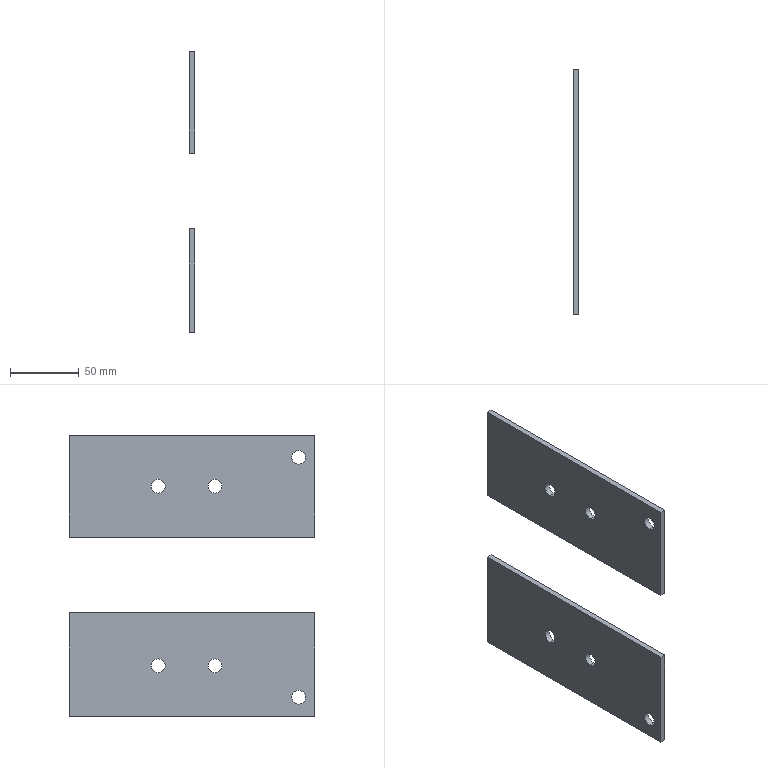Component | SolidWorks | Part2^Assembly2-1 | 2 solids | 24 faces | box 4 x 177.92 x 204 mm | volume 104314 mm3 | cylinder 12 | plane 12 | commonest cylinder face diameters 10 x12
STEP:
#1=COLOUR_RGB('',0.7922,0.8196,0.9333);
#2=FILL_AREA_STYLE_COLOUR('',#1);
#3=FILL_AREA_STYLE('',(#2));
#4=SURFACE_STYLE_FILL_AREA(#3);
#5=SURFACE_SIDE_STYLE('',(#4));
#6=SURFACE_STYLE_USAGE(.BOTH.,#5);
#7=PRESENTATION_STYLE_ASSIGNMENT((#6));
#8=CARTESIAN_POINT('',(6.188,14.393,-35.682));
#9=VERTEX_POINT('',#8);
#10=CARTESIAN_POINT('',(6.188,14.393,-36.076));
#11=VERTEX_POINT('',#10);
#12=CARTESIAN_POINT('',(6.188,14.393,-35.879));
#13=DIRECTION('',(1.,0.,0.));
#14=DIRECTION('',(0.,0.,-1.));
#15=AXIS2_PLACEMENT_3D('',#12,#13,#14);
#16=CIRCLE('',#15,0.1969);
#17=EDGE_CURVE('',#9,#11,#16,.T.);
#18=ORIENTED_EDGE('',*,*,#17,.F.);
#19=CARTESIAN_POINT('',(6.346,14.393,-35.682));
#20=VERTEX_POINT('',#19);
#21=CARTESIAN_POINT('',(2.133,14.393,-35.682));
#22=DIRECTION('',(1.,0.,0.));
#23=VECTOR('',#22,39.37);
#24=LINE('',#21,#23);
#25=EDGE_CURVE('',#9,#20,#24,.T.);
#26=ORIENTED_EDGE('',*,*,#25,.T.);
#27=CARTESIAN_POINT('',(6.346,14.393,-36.076));
#28=VERTEX_POINT('',#27);
#29=CARTESIAN_POINT('',(6.346,14.393,-35.879));
#30=DIRECTION('',(1.,0.,0.));
#31=DIRECTION('',(0.,0.,-1.));
#32=AXIS2_PLACEMENT_3D('',#29,#30,#31);
#33=CIRCLE('',#32,0.1969);
#34=EDGE_CURVE('',#20,#28,#33,.T.);
#35=ORIENTED_EDGE('',*,*,#34,.T.);
#36=CARTESIAN_POINT('',(2.133,14.393,-36.076));
#37=DIRECTION('',(1.,0.,0.));
#38=VECTOR('',#37,39.37);
#39=LINE('',#36,#38);
#40=EDGE_CURVE('',#11,#28,#39,.T.);
#41=ORIENTED_EDGE('',*,*,#40,.F.);
#42=EDGE_LOOP('',(#18,#26,#35,#41));
#43=FACE_OUTER_BOUND('',#42,.T.);
#44=CARTESIAN_POINT('',(2.133,14.393,-35.879));
#45=DIRECTION('',(1.,0.,0.));
#46=DIRECTION('',(0.,0.,-1.));
#47=AXIS2_PLACEMENT_3D('',#44,#45,#46);
#48=CYLINDRICAL_SURFACE('',#47,0.1969);
#49=ADVANCED_FACE('',(#43),#48,.F.);
#50=CARTESIAN_POINT('',(6.188,12.769,-35.682));
#51=VERTEX_POINT('',#50);
#52=CARTESIAN_POINT('',(6.188,12.769,-36.076));
#53=VERTEX_POINT('',#52);
#54=CARTESIAN_POINT('',(6.188,12.769,-35.879));
#55=DIRECTION('',(1.,0.,0.));
#56=DIRECTION('',(0.,0.,-1.));
#57=AXIS2_PLACEMENT_3D('',#54,#55,#56);
#58=CIRCLE('',#57,0.1969);
#59=EDGE_CURVE('',#51,#53,#58,.T.);
#60=ORIENTED_EDGE('',*,*,#59,.F.);
#61=CARTESIAN_POINT('',(6.346,12.769,-35.682));
#62=VERTEX_POINT('',#61);
#63=CARTESIAN_POINT('',(2.133,12.769,-35.682));
#64=DIRECTION('',(1.,0.,0.));
#65=VECTOR('',#64,39.37);
#66=LINE('',#63,#65);
#67=EDGE_CURVE('',#51,#62,#66,.T.);
#68=ORIENTED_EDGE('',*,*,#67,.T.);
#69=CARTESIAN_POINT('',(6.346,12.769,-36.076));
#70=VERTEX_POINT('',#69);
#71=CARTESIAN_POINT('',(6.346,12.769,-35.879));
#72=DIRECTION('',(1.,0.,0.));
#73=DIRECTION('',(0.,0.,-1.));
#74=AXIS2_PLACEMENT_3D('',#71,#72,#73);
#75=CIRCLE('',#74,0.1969);
#76=EDGE_CURVE('',#62,#70,#75,.T.);
#77=ORIENTED_EDGE('',*,*,#76,.T.);
#78=CARTESIAN_POINT('',(2.133,12.769,-36.076));
#79=DIRECTION('',(1.,0.,0.));
#80=VECTOR('',#79,39.37);
#81=LINE('',#78,#80);
#82=EDGE_CURVE('',#53,#70,#81,.T.);
#83=ORIENTED_EDGE('',*,*,#82,.F.);
#84=EDGE_LOOP('',(#60,#68,#77,#83));
#85=FACE_OUTER_BOUND('',#84,.T.);
#86=CARTESIAN_POINT('',(2.133,12.769,-35.879));
#87=DIRECTION('',(1.,0.,0.));
#88=DIRECTION('',(0.,0.,-1.));
#89=AXIS2_PLACEMENT_3D('',#86,#87,#88);
#90=CYLINDRICAL_SURFACE('',#89,0.1969);
#91=ADVANCED_FACE('',(#85),#90,.F.);
#92=CARTESIAN_POINT('',(6.188,10.383,-34.854));
#93=VERTEX_POINT('',#92);
#94=CARTESIAN_POINT('',(6.188,10.383,-35.248));
#95=VERTEX_POINT('',#94);
#96=CARTESIAN_POINT('',(6.188,10.383,-35.051));
#97=DIRECTION('',(1.,0.,0.));
#98=DIRECTION('',(0.,0.,-1.));
#99=AXIS2_PLACEMENT_3D('',#96,#97,#98);
#100=CIRCLE('',#99,0.1969);
#101=EDGE_CURVE('',#93,#95,#100,.T.);
#102=ORIENTED_EDGE('',*,*,#101,.F.);
#103=CARTESIAN_POINT('',(6.346,10.383,-34.854));
#104=VERTEX_POINT('',#103);
#105=CARTESIAN_POINT('',(6.188,10.383,-34.854));
#106=DIRECTION('',(1.,0.,0.));
#107=VECTOR('',#106,39.37);
#108=LINE('',#105,#107);
#109=EDGE_CURVE('',#93,#104,#108,.T.);
#110=ORIENTED_EDGE('',*,*,#109,.T.);
#111=CARTESIAN_POINT('',(6.346,10.383,-35.248));
#112=VERTEX_POINT('',#111);
#113=CARTESIAN_POINT('',(6.346,10.383,-35.051));
#114=DIRECTION('',(1.,0.,0.));
#115=DIRECTION('',(0.,0.,-1.));
#116=AXIS2_PLACEMENT_3D('',#113,#114,#115);
#117=CIRCLE('',#116,0.1969);
#118=EDGE_CURVE('',#104,#112,#117,.T.);
#119=ORIENTED_EDGE('',*,*,#118,.T.);
#120=CARTESIAN_POINT('',(6.188,10.383,-35.248));
#121=DIRECTION('',(1.,0.,0.));
#122=VECTOR('',#121,39.37);
#123=LINE('',#120,#122);
#124=EDGE_CURVE('',#95,#112,#123,.T.);
#125=ORIENTED_EDGE('',*,*,#124,.F.);
#126=EDGE_LOOP('',(#102,#110,#119,#125));
#127=FACE_OUTER_BOUND('',#126,.T.);
#128=CARTESIAN_POINT('',(6.188,10.383,-35.051));
#129=DIRECTION('',(1.,0.,0.));
#130=DIRECTION('',(0.,0.,-1.));
#131=AXIS2_PLACEMENT_3D('',#128,#129,#130);
#132=CYLINDRICAL_SURFACE('',#131,0.1969);
#133=ADVANCED_FACE('',(#127),#132,.F.);
#134=CARTESIAN_POINT('',(6.188,9.924,-34.426));
#135=VERTEX_POINT('',#134);
#136=CARTESIAN_POINT('',(6.188,9.924,-37.333));
#137=VERTEX_POINT('',#136);
#138=CARTESIAN_POINT('',(6.188,9.924,-34.426));
#139=DIRECTION('',(0.,0.,-1.));
#140=VECTOR('',#139,39.37);
#141=LINE('',#138,#140);
#142=EDGE_CURVE('',#135,#137,#141,.T.);
#143=ORIENTED_EDGE('',*,*,#142,.T.);
#144=CARTESIAN_POINT('',(6.346,9.924,-37.333));
#145=VERTEX_POINT('',#144);
#146=CARTESIAN_POINT('',(6.346,9.924,-37.333));
#147=DIRECTION('',(1.,0.,0.));
#148=VECTOR('',#147,39.37);
#149=LINE('',#146,#148);
#150=EDGE_CURVE('',#137,#145,#149,.T.);
#151=ORIENTED_EDGE('',*,*,#150,.T.);
#152=CARTESIAN_POINT('',(6.346,9.924,-34.426));
#153=VERTEX_POINT('',#152);
#154=CARTESIAN_POINT('',(6.346,9.924,-34.426));
#155=DIRECTION('',(0.,0.,-1.));
#156=VECTOR('',#155,39.37);
#157=LINE('',#154,#156);
#158=EDGE_CURVE('',#153,#145,#157,.T.);
#159=ORIENTED_EDGE('',*,*,#158,.F.);
#160=CARTESIAN_POINT('',(6.346,9.924,-34.426));
#161=DIRECTION('',(-1.,-0.,-0.));
#162=VECTOR('',#161,39.37);
#163=LINE('',#160,#162);
#164=EDGE_CURVE('',#153,#135,#163,.T.);
#165=ORIENTED_EDGE('',*,*,#164,.T.);
#166=EDGE_LOOP('',(#143,#151,#159,#165));
#167=FACE_OUTER_BOUND('',#166,.T.);
#168=CARTESIAN_POINT('',(6.346,9.924,-34.426));
#169=DIRECTION('',(-0.,1.,0.));
#170=DIRECTION('',(1.,0.,0.));
#171=AXIS2_PLACEMENT_3D('',#168,#169,#170);
#172=PLANE('',#171);
#173=ADVANCED_FACE('',(#167),#172,.F.);
#174=CARTESIAN_POINT('',(6.346,16.929,-37.333));
#175=VERTEX_POINT('',#174);
#176=CARTESIAN_POINT('',(6.346,16.929,-34.426));
#177=VERTEX_POINT('',#176);
#178=CARTESIAN_POINT('',(6.346,16.929,-34.426));
#179=DIRECTION('',(-0.,-0.,1.));
#180=VECTOR('',#179,39.37);
#181=LINE('',#178,#180);
#182=EDGE_CURVE('',#175,#177,#181,.T.);
#183=ORIENTED_EDGE('',*,*,#182,.F.);
#184=CARTESIAN_POINT('',(6.188,16.929,-37.333));
#185=VERTEX_POINT('',#184);
#186=CARTESIAN_POINT('',(6.346,16.929,-37.333));
#187=DIRECTION('',(-1.,-0.,-0.));
#188=VECTOR('',#187,39.37);
#189=LINE('',#186,#188);
#190=EDGE_CURVE('',#175,#185,#189,.T.);
#191=ORIENTED_EDGE('',*,*,#190,.T.);
#192=CARTESIAN_POINT('',(6.188,16.929,-34.426));
#193=VERTEX_POINT('',#192);
#194=CARTESIAN_POINT('',(6.188,16.929,-34.426));
#195=DIRECTION('',(-0.,-0.,1.));
#196=VECTOR('',#195,39.37);
#197=LINE('',#194,#196);
#198=EDGE_CURVE('',#185,#193,#197,.T.);
#199=ORIENTED_EDGE('',*,*,#198,.T.);
#200=CARTESIAN_POINT('',(6.346,16.929,-34.426));
#201=DIRECTION('',(-1.,-0.,-0.));
#202=VECTOR('',#201,39.37);
#203=LINE('',#200,#202);
#204=EDGE_CURVE('',#177,#193,#203,.T.);
#205=ORIENTED_EDGE('',*,*,#204,.F.);
#206=EDGE_LOOP('',(#183,#191,#199,#205));
#207=FACE_OUTER_BOUND('',#206,.T.);
#208=CARTESIAN_POINT('',(6.346,16.929,-34.426));
#209=DIRECTION('',(0.,-1.,0.));
#210=DIRECTION('',(-1.,-0.,-0.));
#211=AXIS2_PLACEMENT_3D('',#208,#209,#210);
#212=PLANE('',#211);
#213=ADVANCED_FACE('',(#207),#212,.F.);
#214=CARTESIAN_POINT('',(6.346,14.393,-35.879));
#215=DIRECTION('',(1.,0.,0.));
#216=DIRECTION('',(0.,0.,-1.));
#217=AXIS2_PLACEMENT_3D('',#214,#215,#216);
#218=CIRCLE('',#217,0.1969);
#219=EDGE_CURVE('',#28,#20,#218,.T.);
#220=ORIENTED_EDGE('',*,*,#219,.F.);
#221=ORIENTED_EDGE('',*,*,#34,.F.);
#222=EDGE_LOOP('',(#220,#221));
#223=FACE_BOUND('',#222,.T.);
#224=CARTESIAN_POINT('',(6.346,12.769,-35.879));
#225=DIRECTION('',(1.,0.,0.));
#226=DIRECTION('',(0.,0.,-1.));
#227=AXIS2_PLACEMENT_3D('',#224,#225,#226);
#228=CIRCLE('',#227,0.1969);
#229=EDGE_CURVE('',#70,#62,#228,.T.);
#230=ORIENTED_EDGE('',*,*,#229,.F.);
#231=ORIENTED_EDGE('',*,*,#76,.F.);
#232=EDGE_LOOP('',(#230,#231));
#233=FACE_BOUND('',#232,.T.);
#234=CARTESIAN_POINT('',(6.346,17.073,-37.333));
#235=DIRECTION('',(0.,-1.,0.));
#236=VECTOR('',#235,39.37);
#237=LINE('',#234,#236);
#238=EDGE_CURVE('',#175,#145,#237,.T.);
#239=ORIENTED_EDGE('',*,*,#238,.F.);
#240=ORIENTED_EDGE('',*,*,#182,.T.);
#241=CARTESIAN_POINT('',(6.346,16.929,-34.426));
#242=DIRECTION('',(0.,-1.,0.));
#243=VECTOR('',#242,39.37);
#244=LINE('',#241,#243);
#245=EDGE_CURVE('',#177,#153,#244,.T.);
#246=ORIENTED_EDGE('',*,*,#245,.T.);
#247=ORIENTED_EDGE('',*,*,#158,.T.);
#248=EDGE_LOOP('',(#239,#240,#246,#247));
#249=FACE_OUTER_BOUND('',#248,.T.);
#250=CARTESIAN_POINT('',(6.346,10.383,-35.051));
#251=DIRECTION('',(1.,0.,0.));
#252=DIRECTION('',(0.,0.,-1.));
#253=AXIS2_PLACEMENT_3D('',#250,#251,#252);
#254=CIRCLE('',#253,0.1969);
#255=EDGE_CURVE('',#112,#104,#254,.T.);
#256=ORIENTED_EDGE('',*,*,#255,.F.);
#257=ORIENTED_EDGE('',*,*,#118,.F.);
#258=EDGE_LOOP('',(#256,#257));
#259=FACE_BOUND('',#258,.T.);
#260=CARTESIAN_POINT('',(6.346,4.425,-14.841));
#261=DIRECTION('',(1.,0.,0.));
#262=DIRECTION('',(0.,0.,-1.));
#263=AXIS2_PLACEMENT_3D('',#260,#261,#262);
#264=PLANE('',#263);
#265=ADVANCED_FACE('',(#223,#233,#249,#259),#264,.T.);
#266=CARTESIAN_POINT('',(6.188,14.393,-35.879));
#267=DIRECTION('',(1.,0.,0.));
#268=DIRECTION('',(0.,0.,-1.));
#269=AXIS2_PLACEMENT_3D('',#266,#267,#268);
#270=CIRCLE('',#269,0.1969);
#271=EDGE_CURVE('',#11,#9,#270,.T.);
#272=ORIENTED_EDGE('',*,*,#271,.T.);
#273=ORIENTED_EDGE('',*,*,#17,.T.);
#274=EDGE_LOOP('',(#272,#273));
#275=FACE_BOUND('',#274,.T.);
#276=CARTESIAN_POINT('',(6.188,12.769,-35.879));
#277=DIRECTION('',(1.,0.,0.));
#278=DIRECTION('',(0.,0.,-1.));
#279=AXIS2_PLACEMENT_3D('',#276,#277,#278);
#280=CIRCLE('',#279,0.1969);
#281=EDGE_CURVE('',#53,#51,#280,.T.);
#282=ORIENTED_EDGE('',*,*,#281,.T.);
#283=ORIENTED_EDGE('',*,*,#59,.T.);
#284=EDGE_LOOP('',(#282,#283));
#285=FACE_BOUND('',#284,.T.);
#286=CARTESIAN_POINT('',(6.188,10.383,-35.051));
#287=DIRECTION('',(1.,0.,0.));
#288=DIRECTION('',(0.,0.,-1.));
#289=AXIS2_PLACEMENT_3D('',#286,#287,#288);
#290=CIRCLE('',#289,0.1969);
#291=EDGE_CURVE('',#95,#93,#290,.T.);
#292=ORIENTED_EDGE('',*,*,#291,.T.);
#293=ORIENTED_EDGE('',*,*,#101,.T.);
#294=EDGE_LOOP('',(#292,#293));
#295=FACE_BOUND('',#294,.T.);
#296=ORIENTED_EDGE('',*,*,#198,.F.);
#297=CARTESIAN_POINT('',(6.188,4.425,-37.333));
#298=DIRECTION('',(0.,-1.,0.));
#299=VECTOR('',#298,39.37);
#300=LINE('',#297,#299);
#301=EDGE_CURVE('',#185,#137,#300,.T.);
#302=ORIENTED_EDGE('',*,*,#301,.T.);
#303=ORIENTED_EDGE('',*,*,#142,.F.);
#304=CARTESIAN_POINT('',(6.188,16.929,-34.426));
#305=DIRECTION('',(0.,-1.,0.));
#306=VECTOR('',#305,39.37);
#307=LINE('',#304,#306);
#308=EDGE_CURVE('',#193,#135,#307,.T.);
#309=ORIENTED_EDGE('',*,*,#308,.F.);
#310=EDGE_LOOP('',(#296,#302,#303,#309));
#311=FACE_OUTER_BOUND('',#310,.T.);
#312=CARTESIAN_POINT('',(6.188,4.425,-14.841));
#313=DIRECTION('',(1.,0.,0.));
#314=DIRECTION('',(0.,0.,-1.));
#315=AXIS2_PLACEMENT_3D('',#312,#313,#314);
#316=PLANE('',#315);
#317=ADVANCED_FACE('',(#275,#285,#295,#311),#316,.F.);
#318=ORIENTED_EDGE('',*,*,#308,.T.);
#319=ORIENTED_EDGE('',*,*,#164,.F.);
#320=ORIENTED_EDGE('',*,*,#245,.F.);
#321=ORIENTED_EDGE('',*,*,#204,.T.);
#322=EDGE_LOOP('',(#318,#319,#320,#321));
#323=FACE_OUTER_BOUND('',#322,.T.);
#324=CARTESIAN_POINT('',(6.346,16.929,-34.426));
#325=DIRECTION('',(0.,0.,-1.));
#326=DIRECTION('',(-1.,-0.,-0.));
#327=AXIS2_PLACEMENT_3D('',#324,#325,#326);
#328=PLANE('',#327);
#329=ADVANCED_FACE('',(#323),#328,.F.);
#330=ORIENTED_EDGE('',*,*,#109,.F.);
#331=ORIENTED_EDGE('',*,*,#291,.F.);
#332=ORIENTED_EDGE('',*,*,#124,.T.);
#333=ORIENTED_EDGE('',*,*,#255,.T.);
#334=EDGE_LOOP('',(#330,#331,#332,#333));
#335=FACE_OUTER_BOUND('',#334,.T.);
#336=CARTESIAN_POINT('',(6.188,10.383,-35.051));
#337=DIRECTION('',(1.,0.,0.));
#338=DIRECTION('',(0.,0.,-1.));
#339=AXIS2_PLACEMENT_3D('',#336,#337,#338);
#340=CYLINDRICAL_SURFACE('',#339,0.1969);
#341=ADVANCED_FACE('',(#335),#340,.F.);
#342=ORIENTED_EDGE('',*,*,#301,.F.);
#343=ORIENTED_EDGE('',*,*,#190,.F.);
#344=ORIENTED_EDGE('',*,*,#238,.T.);
#345=ORIENTED_EDGE('',*,*,#150,.F.);
#346=EDGE_LOOP('',(#342,#343,#344,#345));
#347=FACE_OUTER_BOUND('',#346,.T.);
#348=CARTESIAN_POINT('',(2.133,17.073,-37.333));
#349=DIRECTION('',(-0.,-0.,1.));
#350=DIRECTION('',(1.,0.,0.));
#351=AXIS2_PLACEMENT_3D('',#348,#349,#350);
#352=PLANE('',#351);
#353=ADVANCED_FACE('',(#347),#352,.F.);
#354=ORIENTED_EDGE('',*,*,#67,.F.);
#355=ORIENTED_EDGE('',*,*,#281,.F.);
#356=ORIENTED_EDGE('',*,*,#82,.T.);
#357=ORIENTED_EDGE('',*,*,#229,.T.);
#358=EDGE_LOOP('',(#354,#355,#356,#357));
#359=FACE_OUTER_BOUND('',#358,.T.);
#360=CARTESIAN_POINT('',(2.133,12.769,-35.879));
#361=DIRECTION('',(1.,0.,0.));
#362=DIRECTION('',(0.,0.,-1.));
#363=AXIS2_PLACEMENT_3D('',#360,#361,#362);
#364=CYLINDRICAL_SURFACE('',#363,0.1969);
#365=ADVANCED_FACE('',(#359),#364,.F.);
#366=ORIENTED_EDGE('',*,*,#25,.F.);
#367=ORIENTED_EDGE('',*,*,#271,.F.);
#368=ORIENTED_EDGE('',*,*,#40,.T.);
#369=ORIENTED_EDGE('',*,*,#219,.T.);
#370=EDGE_LOOP('',(#366,#367,#368,#369));
#371=FACE_OUTER_BOUND('',#370,.T.);
#372=CARTESIAN_POINT('',(2.133,14.393,-35.879));
#373=DIRECTION('',(1.,0.,0.));
#374=DIRECTION('',(0.,0.,-1.));
#375=AXIS2_PLACEMENT_3D('',#372,#373,#374);
#376=CYLINDRICAL_SURFACE('',#375,0.1969);
#377=ADVANCED_FACE('',(#371),#376,.F.);
#378=CLOSED_SHELL('',(#49,#91,#133,#173,#213,#265,#317,#329,#341,#353,#365,#377));
#379=MANIFOLD_SOLID_BREP('',#378);
#380=STYLED_ITEM('',(#7),#379);
#381=(LENGTH_UNIT()NAMED_UNIT(*)SI_UNIT($,.METRE.));
#382=LENGTH_MEASURE_WITH_UNIT(LENGTH_MEASURE(0.0254),#381);
#383=DIMENSIONAL_EXPONENTS(1.,0.,0.,0.,0.,0.,0.);
#384=(CONVERSION_BASED_UNIT('',#382)LENGTH_UNIT()NAMED_UNIT(#383));
#385=UNCERTAINTY_MEASURE_WITH_UNIT(LENGTH_MEASURE(0.00001),#384,'','');
#386=(NAMED_UNIT(*)PLANE_ANGLE_UNIT()SI_UNIT($,.RADIAN.));
#387=(NAMED_UNIT(*)SI_UNIT($,.STERADIAN.)SOLID_ANGLE_UNIT());
#388=(GEOMETRIC_REPRESENTATION_CONTEXT(3)GLOBAL_UNCERTAINTY_ASSIGNED_CONTEXT((#385))GLOBAL_UNIT_ASSIGNED_CONTEXT((#384,#386,#387))REPRESENTATION_CONTEXT('',''));
#389=MECHANICAL_DESIGN_GEOMETRIC_PRESENTATION_REPRESENTATION('',(#380),#388);
#390=PRESENTATION_LAYER_ASSIGNMENT('','',(#380));
#391=COLOUR_RGB('',0.7922,0.8196,0.9333);
#392=FILL_AREA_STYLE_COLOUR('',#391);
#393=FILL_AREA_STYLE('',(#392));
#394=SURFACE_STYLE_FILL_AREA(#393);
#395=SURFACE_SIDE_STYLE('',(#394));
#396=SURFACE_STYLE_USAGE(.BOTH.,#395);
#397=PRESENTATION_STYLE_ASSIGNMENT((#396));
#398=CARTESIAN_POINT('',(6.188,12.769,-40.807));
#399=VERTEX_POINT('',#398);
#400=CARTESIAN_POINT('',(6.188,12.769,-41.201));
#401=VERTEX_POINT('',#400);
#402=CARTESIAN_POINT('',(6.188,12.769,-41.004));
#403=DIRECTION('',(1.,0.,0.));
#404=DIRECTION('',(0.,0.,-1.));
#405=AXIS2_PLACEMENT_3D('',#402,#403,#404);
#406=CIRCLE('',#405,0.1969);
#407=EDGE_CURVE('',#399,#401,#406,.T.);
#408=ORIENTED_EDGE('',*,*,#407,.F.);
#409=CARTESIAN_POINT('',(6.346,12.769,-40.807));
#410=VERTEX_POINT('',#409);
#411=CARTESIAN_POINT('',(2.133,12.769,-40.807));
#412=DIRECTION('',(1.,0.,0.));
#413=VECTOR('',#412,39.37);
#414=LINE('',#411,#413);
#415=EDGE_CURVE('',#399,#410,#414,.T.);
#416=ORIENTED_EDGE('',*,*,#415,.T.);
#417=CARTESIAN_POINT('',(6.346,12.769,-41.201));
#418=VERTEX_POINT('',#417);
#419=CARTESIAN_POINT('',(6.346,12.769,-41.004));
#420=DIRECTION('',(1.,0.,0.));
#421=DIRECTION('',(0.,0.,1.));
#422=AXIS2_PLACEMENT_3D('',#419,#420,#421);
#423=CIRCLE('',#422,0.1969);
#424=EDGE_CURVE('',#410,#418,#423,.T.);
#425=ORIENTED_EDGE('',*,*,#424,.T.);
#426=CARTESIAN_POINT('',(2.133,12.769,-41.201));
#427=DIRECTION('',(1.,0.,0.));
#428=VECTOR('',#427,39.37);
#429=LINE('',#426,#428);
#430=EDGE_CURVE('',#401,#418,#429,.T.);
#431=ORIENTED_EDGE('',*,*,#430,.F.);
#432=EDGE_LOOP('',(#408,#416,#425,#431));
#433=FACE_OUTER_BOUND('',#432,.T.);
#434=CARTESIAN_POINT('',(2.133,12.769,-41.004));
#435=DIRECTION('',(1.,0.,0.));
#436=DIRECTION('',(0.,0.,-1.));
#437=AXIS2_PLACEMENT_3D('',#434,#435,#436);
#438=CYLINDRICAL_SURFACE('',#437,0.1969);
#439=ADVANCED_FACE('',(#433),#438,.F.);
#440=CARTESIAN_POINT('',(6.188,14.393,-40.807));
#441=VERTEX_POINT('',#440);
#442=CARTESIAN_POINT('',(6.188,14.393,-41.201));
#443=VERTEX_POINT('',#442);
#444=CARTESIAN_POINT('',(6.188,14.393,-41.004));
#445=DIRECTION('',(1.,0.,0.));
#446=DIRECTION('',(0.,0.,-1.));
#447=AXIS2_PLACEMENT_3D('',#444,#445,#446);
#448=CIRCLE('',#447,0.1969);
#449=EDGE_CURVE('',#441,#443,#448,.T.);
#450=ORIENTED_EDGE('',*,*,#449,.F.);
#451=CARTESIAN_POINT('',(6.346,14.393,-40.807));
#452=VERTEX_POINT('',#451);
#453=CARTESIAN_POINT('',(2.133,14.393,-40.807));
#454=DIRECTION('',(1.,0.,0.));
#455=VECTOR('',#454,39.37);
#456=LINE('',#453,#455);
#457=EDGE_CURVE('',#441,#452,#456,.T.);
#458=ORIENTED_EDGE('',*,*,#457,.T.);
#459=CARTESIAN_POINT('',(6.346,14.393,-41.201));
#460=VERTEX_POINT('',#459);
#461=CARTESIAN_POINT('',(6.346,14.393,-41.004));
#462=DIRECTION('',(1.,0.,0.));
#463=DIRECTION('',(0.,0.,1.));
#464=AXIS2_PLACEMENT_3D('',#461,#462,#463);
#465=CIRCLE('',#464,0.1969);
#466=EDGE_CURVE('',#452,#460,#465,.T.);
#467=ORIENTED_EDGE('',*,*,#466,.T.);
#468=CARTESIAN_POINT('',(2.133,14.393,-41.201));
#469=DIRECTION('',(1.,0.,0.));
#470=VECTOR('',#469,39.37);
#471=LINE('',#468,#470);
#472=EDGE_CURVE('',#443,#460,#471,.T.);
#473=ORIENTED_EDGE('',*,*,#472,.F.);
#474=EDGE_LOOP('',(#450,#458,#467,#473));
#475=FACE_OUTER_BOUND('',#474,.T.);
#476=CARTESIAN_POINT('',(2.133,14.393,-41.004));
#477=DIRECTION('',(1.,0.,0.));
#478=DIRECTION('',(0.,0.,-1.));
#479=AXIS2_PLACEMENT_3D('',#476,#477,#478);
#480=CYLINDRICAL_SURFACE('',#479,0.1969);
#481=ADVANCED_FACE('',(#475),#480,.F.);
#482=CARTESIAN_POINT('',(6.188,10.383,-41.704));
#483=VERTEX_POINT('',#482);
#484=CARTESIAN_POINT('',(6.188,10.383,-42.098));
#485=VERTEX_POINT('',#484);
#486=CARTESIAN_POINT('',(6.188,10.383,-41.901));
#487=DIRECTION('',(1.,0.,0.));
#488=DIRECTION('',(0.,0.,-1.));
#489=AXIS2_PLACEMENT_3D('',#486,#487,#488);
#490=CIRCLE('',#489,0.1969);
#491=EDGE_CURVE('',#483,#485,#490,.T.);
#492=ORIENTED_EDGE('',*,*,#491,.F.);
#493=CARTESIAN_POINT('',(6.346,10.383,-41.704));
#494=VERTEX_POINT('',#493);
#495=CARTESIAN_POINT('',(6.188,10.383,-41.704));
#496=DIRECTION('',(1.,0.,0.));
#497=VECTOR('',#496,39.37);
#498=LINE('',#495,#497);
#499=EDGE_CURVE('',#483,#494,#498,.T.);
#500=ORIENTED_EDGE('',*,*,#499,.T.);
#501=CARTESIAN_POINT('',(6.346,10.383,-42.098));
#502=VERTEX_POINT('',#501);
#503=CARTESIAN_POINT('',(6.346,10.383,-41.901));
#504=DIRECTION('',(1.,0.,0.));
#505=DIRECTION('',(0.,0.,-1.));
#506=AXIS2_PLACEMENT_3D('',#503,#504,#505);
#507=CIRCLE('',#506,0.1969);
#508=EDGE_CURVE('',#494,#502,#507,.T.);
#509=ORIENTED_EDGE('',*,*,#508,.T.);
#510=CARTESIAN_POINT('',(6.188,10.383,-42.098));
#511=DIRECTION('',(1.,0.,0.));
#512=VECTOR('',#511,39.37);
#513=LINE('',#510,#512);
#514=EDGE_CURVE('',#485,#502,#513,.T.);
#515=ORIENTED_EDGE('',*,*,#514,.F.);
#516=EDGE_LOOP('',(#492,#500,#509,#515));
#517=FACE_OUTER_BOUND('',#516,.T.);
#518=CARTESIAN_POINT('',(6.188,10.383,-41.901));
#519=DIRECTION('',(1.,0.,0.));
#520=DIRECTION('',(0.,0.,-1.));
#521=AXIS2_PLACEMENT_3D('',#518,#519,#520);
#522=CYLINDRICAL_SURFACE('',#521,0.1969);
#523=ADVANCED_FACE('',(#517),#522,.F.);
#524=CARTESIAN_POINT('',(6.188,9.924,-42.457));
#525=VERTEX_POINT('',#524);
#526=CARTESIAN_POINT('',(6.188,16.929,-42.457));
#527=VERTEX_POINT('',#526);
#528=CARTESIAN_POINT('',(6.188,16.929,-42.457));
#529=DIRECTION('',(-0.,1.,0.));
#530=VECTOR('',#529,39.37);
#531=LINE('',#528,#530);
#532=EDGE_CURVE('',#525,#527,#531,.T.);
#533=ORIENTED_EDGE('',*,*,#532,.T.);
#534=CARTESIAN_POINT('',(6.346,16.929,-42.457));
#535=VERTEX_POINT('',#534);
#536=CARTESIAN_POINT('',(6.346,16.929,-42.457));
#537=DIRECTION('',(-1.,-0.,-0.));
#538=VECTOR('',#537,39.37);
#539=LINE('',#536,#538);
#540=EDGE_CURVE('',#535,#527,#539,.T.);
#541=ORIENTED_EDGE('',*,*,#540,.F.);
#542=CARTESIAN_POINT('',(6.346,9.924,-42.457));
#543=VERTEX_POINT('',#542);
#544=CARTESIAN_POINT('',(6.346,16.929,-42.457));
#545=DIRECTION('',(-0.,1.,0.));
#546=VECTOR('',#545,39.37);
#547=LINE('',#544,#546);
#548=EDGE_CURVE('',#543,#535,#547,.T.);
#549=ORIENTED_EDGE('',*,*,#548,.F.);
#550=CARTESIAN_POINT('',(6.346,9.924,-42.457));
#551=DIRECTION('',(-1.,-0.,-0.));
#552=VECTOR('',#551,39.37);
#553=LINE('',#550,#552);
#554=EDGE_CURVE('',#543,#525,#553,.T.);
#555=ORIENTED_EDGE('',*,*,#554,.T.);
#556=EDGE_LOOP('',(#533,#541,#549,#555));
#557=FACE_OUTER_BOUND('',#556,.T.);
#558=CARTESIAN_POINT('',(6.346,16.929,-42.457));
#559=DIRECTION('',(-0.,-0.,1.));
#560=DIRECTION('',(1.,0.,0.));
#561=AXIS2_PLACEMENT_3D('',#558,#559,#560);
#562=PLANE('',#561);
#563=ADVANCED_FACE('',(#557),#562,.F.);
#564=ORIENTED_EDGE('',*,*,#499,.F.);
#565=CARTESIAN_POINT('',(6.188,10.383,-41.901));
#566=DIRECTION('',(1.,0.,0.));
#567=DIRECTION('',(0.,0.,-1.));
#568=AXIS2_PLACEMENT_3D('',#565,#566,#567);
#569=CIRCLE('',#568,0.1969);
#570=EDGE_CURVE('',#485,#483,#569,.T.);
#571=ORIENTED_EDGE('',*,*,#570,.F.);
#572=ORIENTED_EDGE('',*,*,#514,.T.);
#573=CARTESIAN_POINT('',(6.346,10.383,-41.901));
#574=DIRECTION('',(1.,0.,0.));
#575=DIRECTION('',(0.,0.,-1.));
#576=AXIS2_PLACEMENT_3D('',#573,#574,#575);
#577=CIRCLE('',#576,0.1969);
#578=EDGE_CURVE('',#502,#494,#577,.T.);
#579=ORIENTED_EDGE('',*,*,#578,.T.);
#580=EDGE_LOOP('',(#564,#571,#572,#579));
#581=FACE_OUTER_BOUND('',#580,.T.);
#582=CARTESIAN_POINT('',(6.188,10.383,-41.901));
#583=DIRECTION('',(1.,0.,0.));
#584=DIRECTION('',(0.,0.,-1.));
#585=AXIS2_PLACEMENT_3D('',#582,#583,#584);
#586=CYLINDRICAL_SURFACE('',#585,0.1969);
#587=ADVANCED_FACE('',(#581),#586,.F.);
#588=CARTESIAN_POINT('',(6.346,12.769,-41.004));
#589=DIRECTION('',(1.,0.,0.));
#590=DIRECTION('',(0.,0.,1.));
#591=AXIS2_PLACEMENT_3D('',#588,#589,#590);
#592=CIRCLE('',#591,0.1969);
#593=EDGE_CURVE('',#418,#410,#592,.T.);
#594=ORIENTED_EDGE('',*,*,#593,.F.);
#595=ORIENTED_EDGE('',*,*,#424,.F.);
#596=EDGE_LOOP('',(#594,#595));
#597=FACE_BOUND('',#596,.T.);
#598=CARTESIAN_POINT('',(6.346,14.393,-41.004));
#599=DIRECTION('',(1.,0.,0.));
#600=DIRECTION('',(0.,0.,1.));
#601=AXIS2_PLACEMENT_3D('',#598,#599,#600);
#602=CIRCLE('',#601,0.1969);
#603=EDGE_CURVE('',#460,#452,#602,.T.);
#604=ORIENTED_EDGE('',*,*,#603,.F.);
#605=ORIENTED_EDGE('',*,*,#466,.F.);
#606=EDGE_LOOP('',(#604,#605));
#607=FACE_BOUND('',#606,.T.);
#608=CARTESIAN_POINT('',(6.346,9.924,-39.489));
#609=VERTEX_POINT('',#608);
#610=CARTESIAN_POINT('',(6.346,16.929,-39.489));
#611=VERTEX_POINT('',#610);
#612=CARTESIAN_POINT('',(6.346,17.073,-39.489));
#613=DIRECTION('',(-0.,1.,0.));
#614=VECTOR('',#613,39.37);
#615=LINE('',#612,#614);
#616=EDGE_CURVE('',#609,#611,#615,.T.);
#617=ORIENTED_EDGE('',*,*,#616,.F.);
#618=CARTESIAN_POINT('',(6.346,9.924,-34.426));
#619=DIRECTION('',(0.,0.,-1.));
#620=VECTOR('',#619,39.37);
#621=LINE('',#618,#620);
#622=EDGE_CURVE('',#609,#543,#621,.T.);
#623=ORIENTED_EDGE('',*,*,#622,.T.);
#624=ORIENTED_EDGE('',*,*,#548,.T.);
#625=CARTESIAN_POINT('',(6.346,16.929,-34.426));
#626=DIRECTION('',(-0.,-0.,1.));
#627=VECTOR('',#626,39.37);
#628=LINE('',#625,#627);
#629=EDGE_CURVE('',#535,#611,#628,.T.);
#630=ORIENTED_EDGE('',*,*,#629,.T.);
#631=EDGE_LOOP('',(#617,#623,#624,#630));
#632=FACE_OUTER_BOUND('',#631,.T.);
#633=ORIENTED_EDGE('',*,*,#578,.F.);
#634=ORIENTED_EDGE('',*,*,#508,.F.);
#635=EDGE_LOOP('',(#633,#634));
#636=FACE_BOUND('',#635,.T.);
#637=CARTESIAN_POINT('',(6.346,4.425,-14.841));
#638=DIRECTION('',(1.,0.,0.));
#639=DIRECTION('',(0.,0.,-1.));
#640=AXIS2_PLACEMENT_3D('',#637,#638,#639);
#641=PLANE('',#640);
#642=ADVANCED_FACE('',(#597,#607,#632,#636),#641,.T.);
#643=CARTESIAN_POINT('',(6.188,12.769,-41.004));
#644=DIRECTION('',(1.,0.,0.));
#645=DIRECTION('',(0.,0.,-1.));
#646=AXIS2_PLACEMENT_3D('',#643,#644,#645);
#647=CIRCLE('',#646,0.1969);
#648=EDGE_CURVE('',#401,#399,#647,.T.);
#649=ORIENTED_EDGE('',*,*,#648,.T.);
#650=ORIENTED_EDGE('',*,*,#407,.T.);
#651=EDGE_LOOP('',(#649,#650));
#652=FACE_BOUND('',#651,.T.);
#653=CARTESIAN_POINT('',(6.188,14.393,-41.004));
#654=DIRECTION('',(1.,0.,0.));
#655=DIRECTION('',(0.,0.,-1.));
#656=AXIS2_PLACEMENT_3D('',#653,#654,#655);
#657=CIRCLE('',#656,0.1969);
#658=EDGE_CURVE('',#443,#441,#657,.T.);
#659=ORIENTED_EDGE('',*,*,#658,.T.);
#660=ORIENTED_EDGE('',*,*,#449,.T.);
#661=EDGE_LOOP('',(#659,#660));
#662=FACE_BOUND('',#661,.T.);
#663=ORIENTED_EDGE('',*,*,#570,.T.);
#664=ORIENTED_EDGE('',*,*,#491,.T.);
#665=EDGE_LOOP('',(#663,#664));
#666=FACE_BOUND('',#665,.T.);
#667=CARTESIAN_POINT('',(6.188,9.924,-39.489));
#668=VERTEX_POINT('',#667);
#669=CARTESIAN_POINT('',(6.188,9.924,-34.426));
#670=DIRECTION('',(0.,0.,-1.));
#671=VECTOR('',#670,39.37);
#672=LINE('',#669,#671);
#673=EDGE_CURVE('',#668,#525,#672,.T.);
#674=ORIENTED_EDGE('',*,*,#673,.F.);
#675=CARTESIAN_POINT('',(6.188,16.929,-39.489));
#676=VERTEX_POINT('',#675);
#677=CARTESIAN_POINT('',(6.188,4.425,-39.489));
#678=DIRECTION('',(-0.,1.,0.));
#679=VECTOR('',#678,39.37);
#680=LINE('',#677,#679);
#681=EDGE_CURVE('',#668,#676,#680,.T.);
#682=ORIENTED_EDGE('',*,*,#681,.T.);
#683=CARTESIAN_POINT('',(6.188,16.929,-34.426));
#684=DIRECTION('',(-0.,-0.,1.));
#685=VECTOR('',#684,39.37);
#686=LINE('',#683,#685);
#687=EDGE_CURVE('',#527,#676,#686,.T.);
#688=ORIENTED_EDGE('',*,*,#687,.F.);
#689=ORIENTED_EDGE('',*,*,#532,.F.);
#690=EDGE_LOOP('',(#674,#682,#688,#689));
#691=FACE_OUTER_BOUND('',#690,.T.);
#692=CARTESIAN_POINT('',(6.188,4.425,-14.841));
#693=DIRECTION('',(1.,0.,0.));
#694=DIRECTION('',(0.,0.,-1.));
#695=AXIS2_PLACEMENT_3D('',#692,#693,#694);
#696=PLANE('',#695);
#697=ADVANCED_FACE('',(#652,#662,#666,#691),#696,.F.);
#698=ORIENTED_EDGE('',*,*,#687,.T.);
#699=CARTESIAN_POINT('',(6.346,16.929,-39.489));
#700=DIRECTION('',(1.,0.,0.));
#701=VECTOR('',#700,39.37);
#702=LINE('',#699,#701);
#703=EDGE_CURVE('',#676,#611,#702,.T.);
#704=ORIENTED_EDGE('',*,*,#703,.T.);
#705=ORIENTED_EDGE('',*,*,#629,.F.);
#706=ORIENTED_EDGE('',*,*,#540,.T.);
#707=EDGE_LOOP('',(#698,#704,#705,#706));
#708=FACE_OUTER_BOUND('',#707,.T.);
#709=CARTESIAN_POINT('',(6.346,16.929,-34.426));
#710=DIRECTION('',(0.,-1.,0.));
#711=DIRECTION('',(-1.,-0.,-0.));
#712=AXIS2_PLACEMENT_3D('',#709,#710,#711);
#713=PLANE('',#712);
#714=ADVANCED_FACE('',(#708),#713,.F.);
#715=ORIENTED_EDGE('',*,*,#622,.F.);
#716=CARTESIAN_POINT('',(6.346,9.924,-39.489));
#717=DIRECTION('',(-1.,-0.,-0.));
#718=VECTOR('',#717,39.37);
#719=LINE('',#716,#718);
#720=EDGE_CURVE('',#609,#668,#719,.T.);
#721=ORIENTED_EDGE('',*,*,#720,.T.);
#722=ORIENTED_EDGE('',*,*,#673,.T.);
#723=ORIENTED_EDGE('',*,*,#554,.F.);
#724=EDGE_LOOP('',(#715,#721,#722,#723));
#725=FACE_OUTER_BOUND('',#724,.T.);
#726=CARTESIAN_POINT('',(6.346,9.924,-34.426));
#727=DIRECTION('',(-0.,1.,0.));
#728=DIRECTION('',(1.,0.,0.));
#729=AXIS2_PLACEMENT_3D('',#726,#727,#728);
#730=PLANE('',#729);
#731=ADVANCED_FACE('',(#725),#730,.F.);
#732=ORIENTED_EDGE('',*,*,#616,.T.);
#733=ORIENTED_EDGE('',*,*,#703,.F.);
#734=ORIENTED_EDGE('',*,*,#681,.F.);
#735=ORIENTED_EDGE('',*,*,#720,.F.);
#736=EDGE_LOOP('',(#732,#733,#734,#735));
#737=FACE_OUTER_BOUND('',#736,.T.);
#738=CARTESIAN_POINT('',(2.133,17.073,-39.489));
#739=DIRECTION('',(0.,0.,-1.));
#740=DIRECTION('',(-1.,-0.,-0.));
#741=AXIS2_PLACEMENT_3D('',#738,#739,#740);
#742=PLANE('',#741);
#743=ADVANCED_FACE('',(#737),#742,.F.);
#744=ORIENTED_EDGE('',*,*,#457,.F.);
#745=ORIENTED_EDGE('',*,*,#658,.F.);
#746=ORIENTED_EDGE('',*,*,#472,.T.);
#747=ORIENTED_EDGE('',*,*,#603,.T.);
#748=EDGE_LOOP('',(#744,#745,#746,#747));
#749=FACE_OUTER_BOUND('',#748,.T.);
#750=CARTESIAN_POINT('',(2.133,14.393,-41.004));
#751=DIRECTION('',(1.,0.,0.));
#752=DIRECTION('',(0.,0.,-1.));
#753=AXIS2_PLACEMENT_3D('',#750,#751,#752);
#754=CYLINDRICAL_SURFACE('',#753,0.1969);
#755=ADVANCED_FACE('',(#749),#754,.F.);
#756=ORIENTED_EDGE('',*,*,#415,.F.);
#757=ORIENTED_EDGE('',*,*,#648,.F.);
#758=ORIENTED_EDGE('',*,*,#430,.T.);
#759=ORIENTED_EDGE('',*,*,#593,.T.);
#760=EDGE_LOOP('',(#756,#757,#758,#759));
#761=FACE_OUTER_BOUND('',#760,.T.);
#762=CARTESIAN_POINT('',(2.133,12.769,-41.004));
#763=DIRECTION('',(1.,0.,0.));
#764=DIRECTION('',(0.,0.,-1.));
#765=AXIS2_PLACEMENT_3D('',#762,#763,#764);
#766=CYLINDRICAL_SURFACE('',#765,0.1969);
#767=ADVANCED_FACE('',(#761),#766,.F.);
#768=CLOSED_SHELL('',(#439,#481,#523,#563,#587,#642,#697,#714,#731,#743,#755,#767));
#769=MANIFOLD_SOLID_BREP('',#768);
#770=STYLED_ITEM('',(#397),#769);
#771=(LENGTH_UNIT()NAMED_UNIT(*)SI_UNIT($,.METRE.));
#772=LENGTH_MEASURE_WITH_UNIT(LENGTH_MEASURE(0.0254),#771);
#773=DIMENSIONAL_EXPONENTS(1.,0.,0.,0.,0.,0.,0.);
#774=(CONVERSION_BASED_UNIT('',#772)LENGTH_UNIT()NAMED_UNIT(#773));
#775=UNCERTAINTY_MEASURE_WITH_UNIT(LENGTH_MEASURE(0.00001),#774,'','');
#776=(NAMED_UNIT(*)PLANE_ANGLE_UNIT()SI_UNIT($,.RADIAN.));
#777=(NAMED_UNIT(*)SI_UNIT($,.STERADIAN.)SOLID_ANGLE_UNIT());
#778=(GEOMETRIC_REPRESENTATION_CONTEXT(3)GLOBAL_UNCERTAINTY_ASSIGNED_CONTEXT((#775))GLOBAL_UNIT_ASSIGNED_CONTEXT((#774,#776,#777))REPRESENTATION_CONTEXT('',''));
#779=MECHANICAL_DESIGN_GEOMETRIC_PRESENTATION_REPRESENTATION('',(#770),#778);
#780=PRESENTATION_LAYER_ASSIGNMENT('','',(#770));
#781=CARTESIAN_POINT('',(0.,0.,0.));
#782=DIRECTION('',(0.,0.,1.));
#783=DIRECTION('',(1.,0.,0.));
#784=AXIS2_PLACEMENT_3D('',#781,#782,#783);
#785=(LENGTH_UNIT()NAMED_UNIT(*)SI_UNIT($,.METRE.));
#786=LENGTH_MEASURE_WITH_UNIT(LENGTH_MEASURE(0.0254),#785);
#787=DIMENSIONAL_EXPONENTS(1.,0.,0.,0.,0.,0.,0.);
#788=(CONVERSION_BASED_UNIT('',#786)LENGTH_UNIT()NAMED_UNIT(#787));
#789=UNCERTAINTY_MEASURE_WITH_UNIT(LENGTH_MEASURE(0.00001),#788,'','');
#790=(NAMED_UNIT(*)PLANE_ANGLE_UNIT()SI_UNIT($,.RADIAN.));
#791=(NAMED_UNIT(*)SI_UNIT($,.STERADIAN.)SOLID_ANGLE_UNIT());
#792=(GEOMETRIC_REPRESENTATION_CONTEXT(3)GLOBAL_UNCERTAINTY_ASSIGNED_CONTEXT((#789))GLOBAL_UNIT_ASSIGNED_CONTEXT((#788,#790,#791))REPRESENTATION_CONTEXT('',''));
#793=ADVANCED_BREP_SHAPE_REPRESENTATION('',(#769,#379,#784),#792);